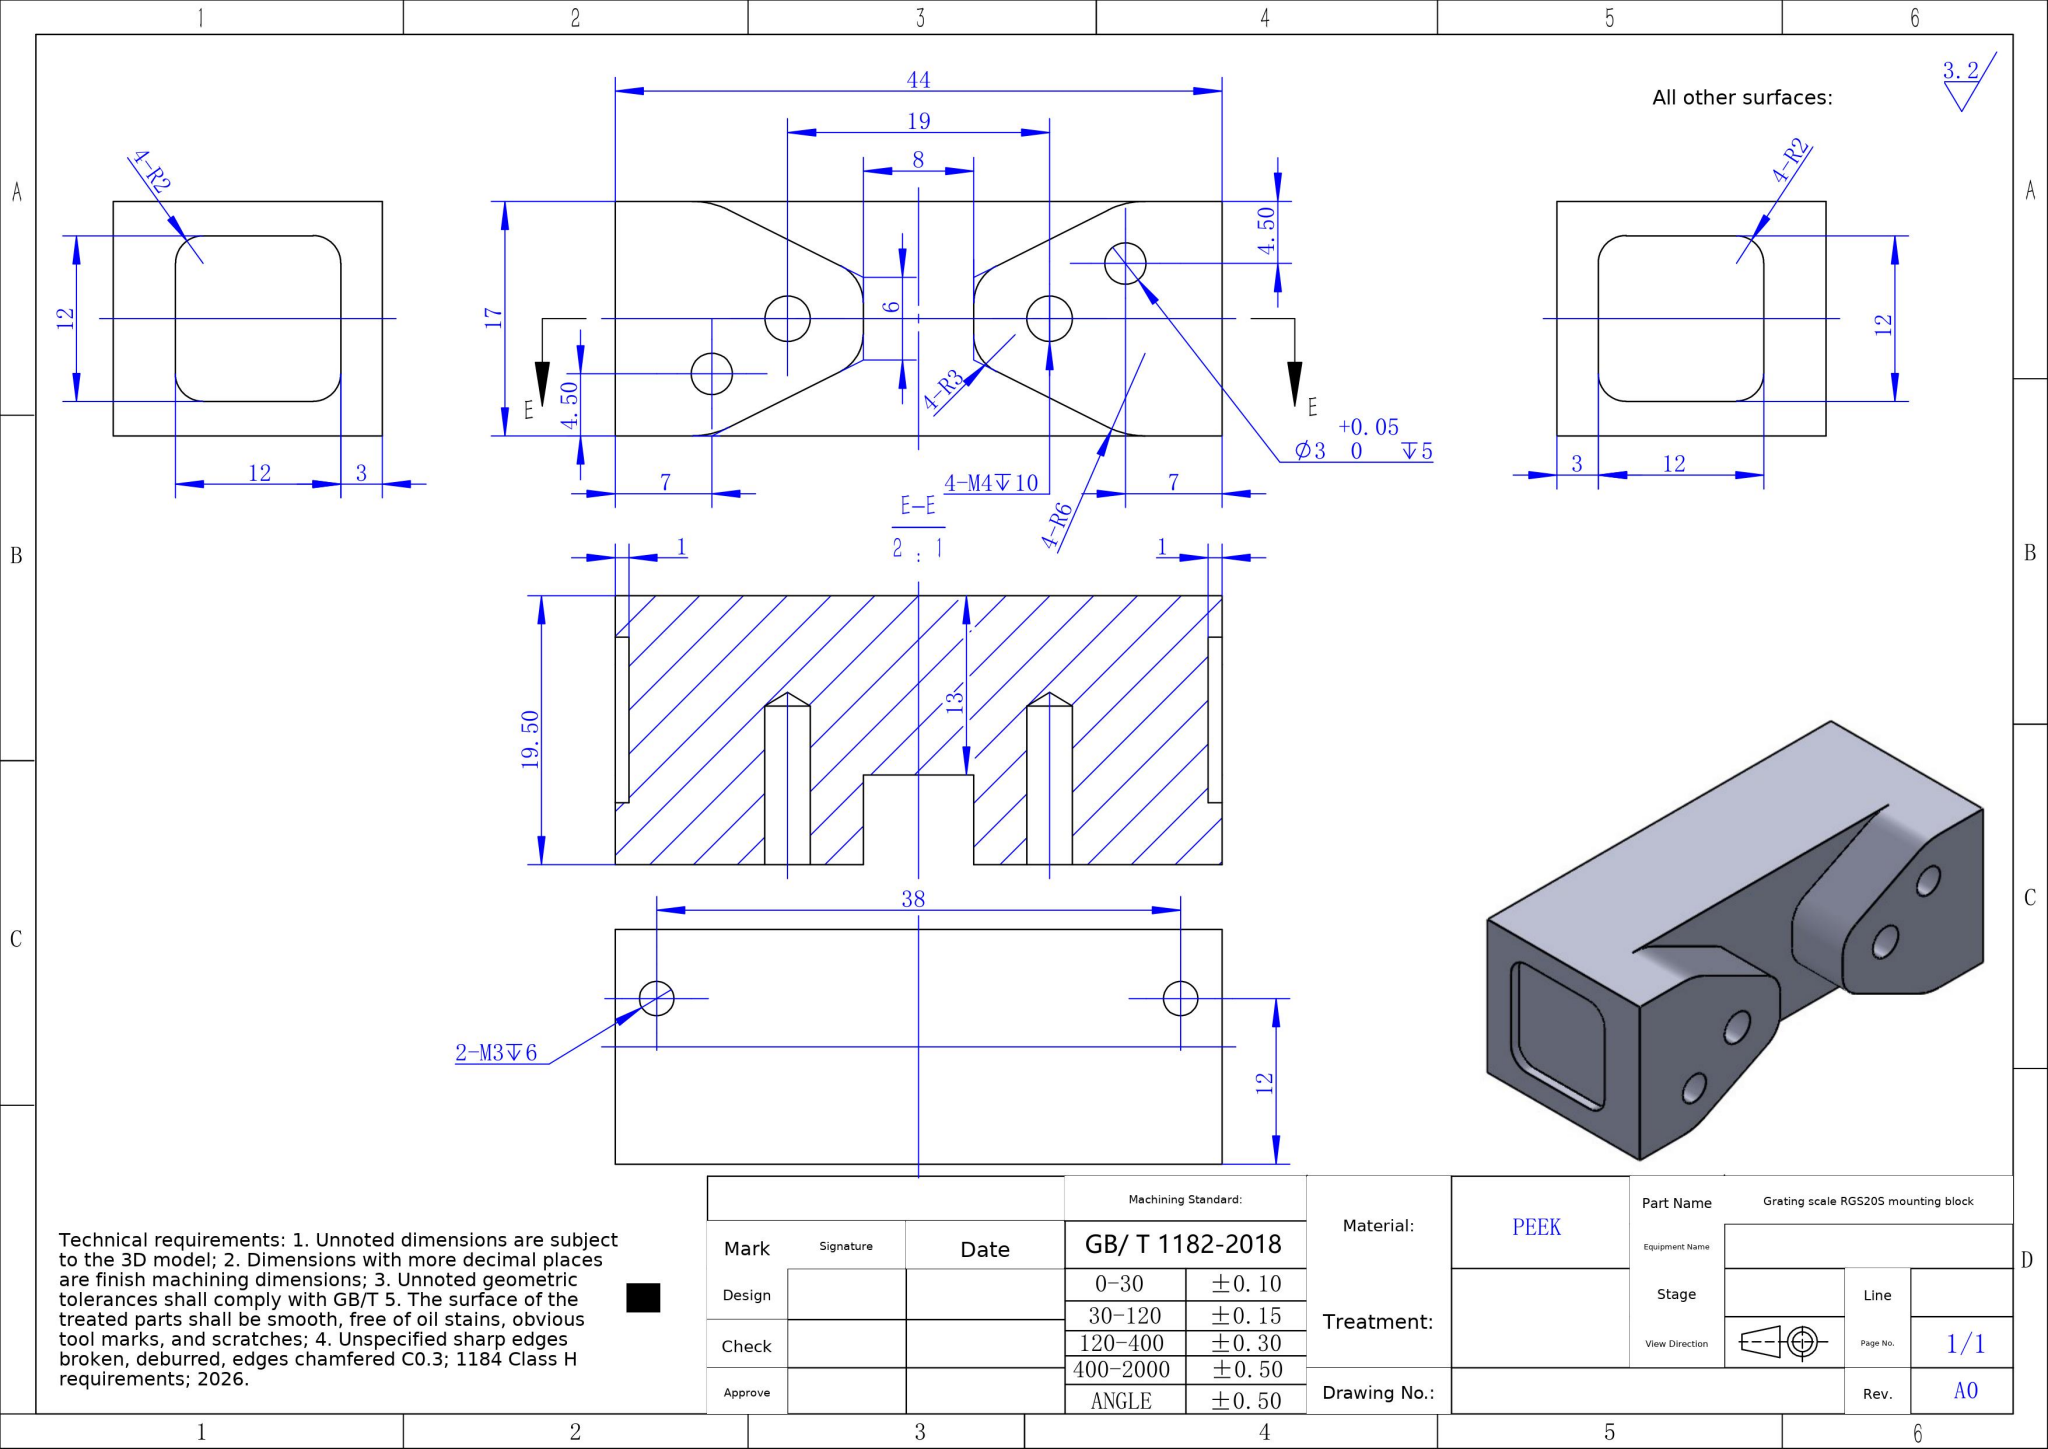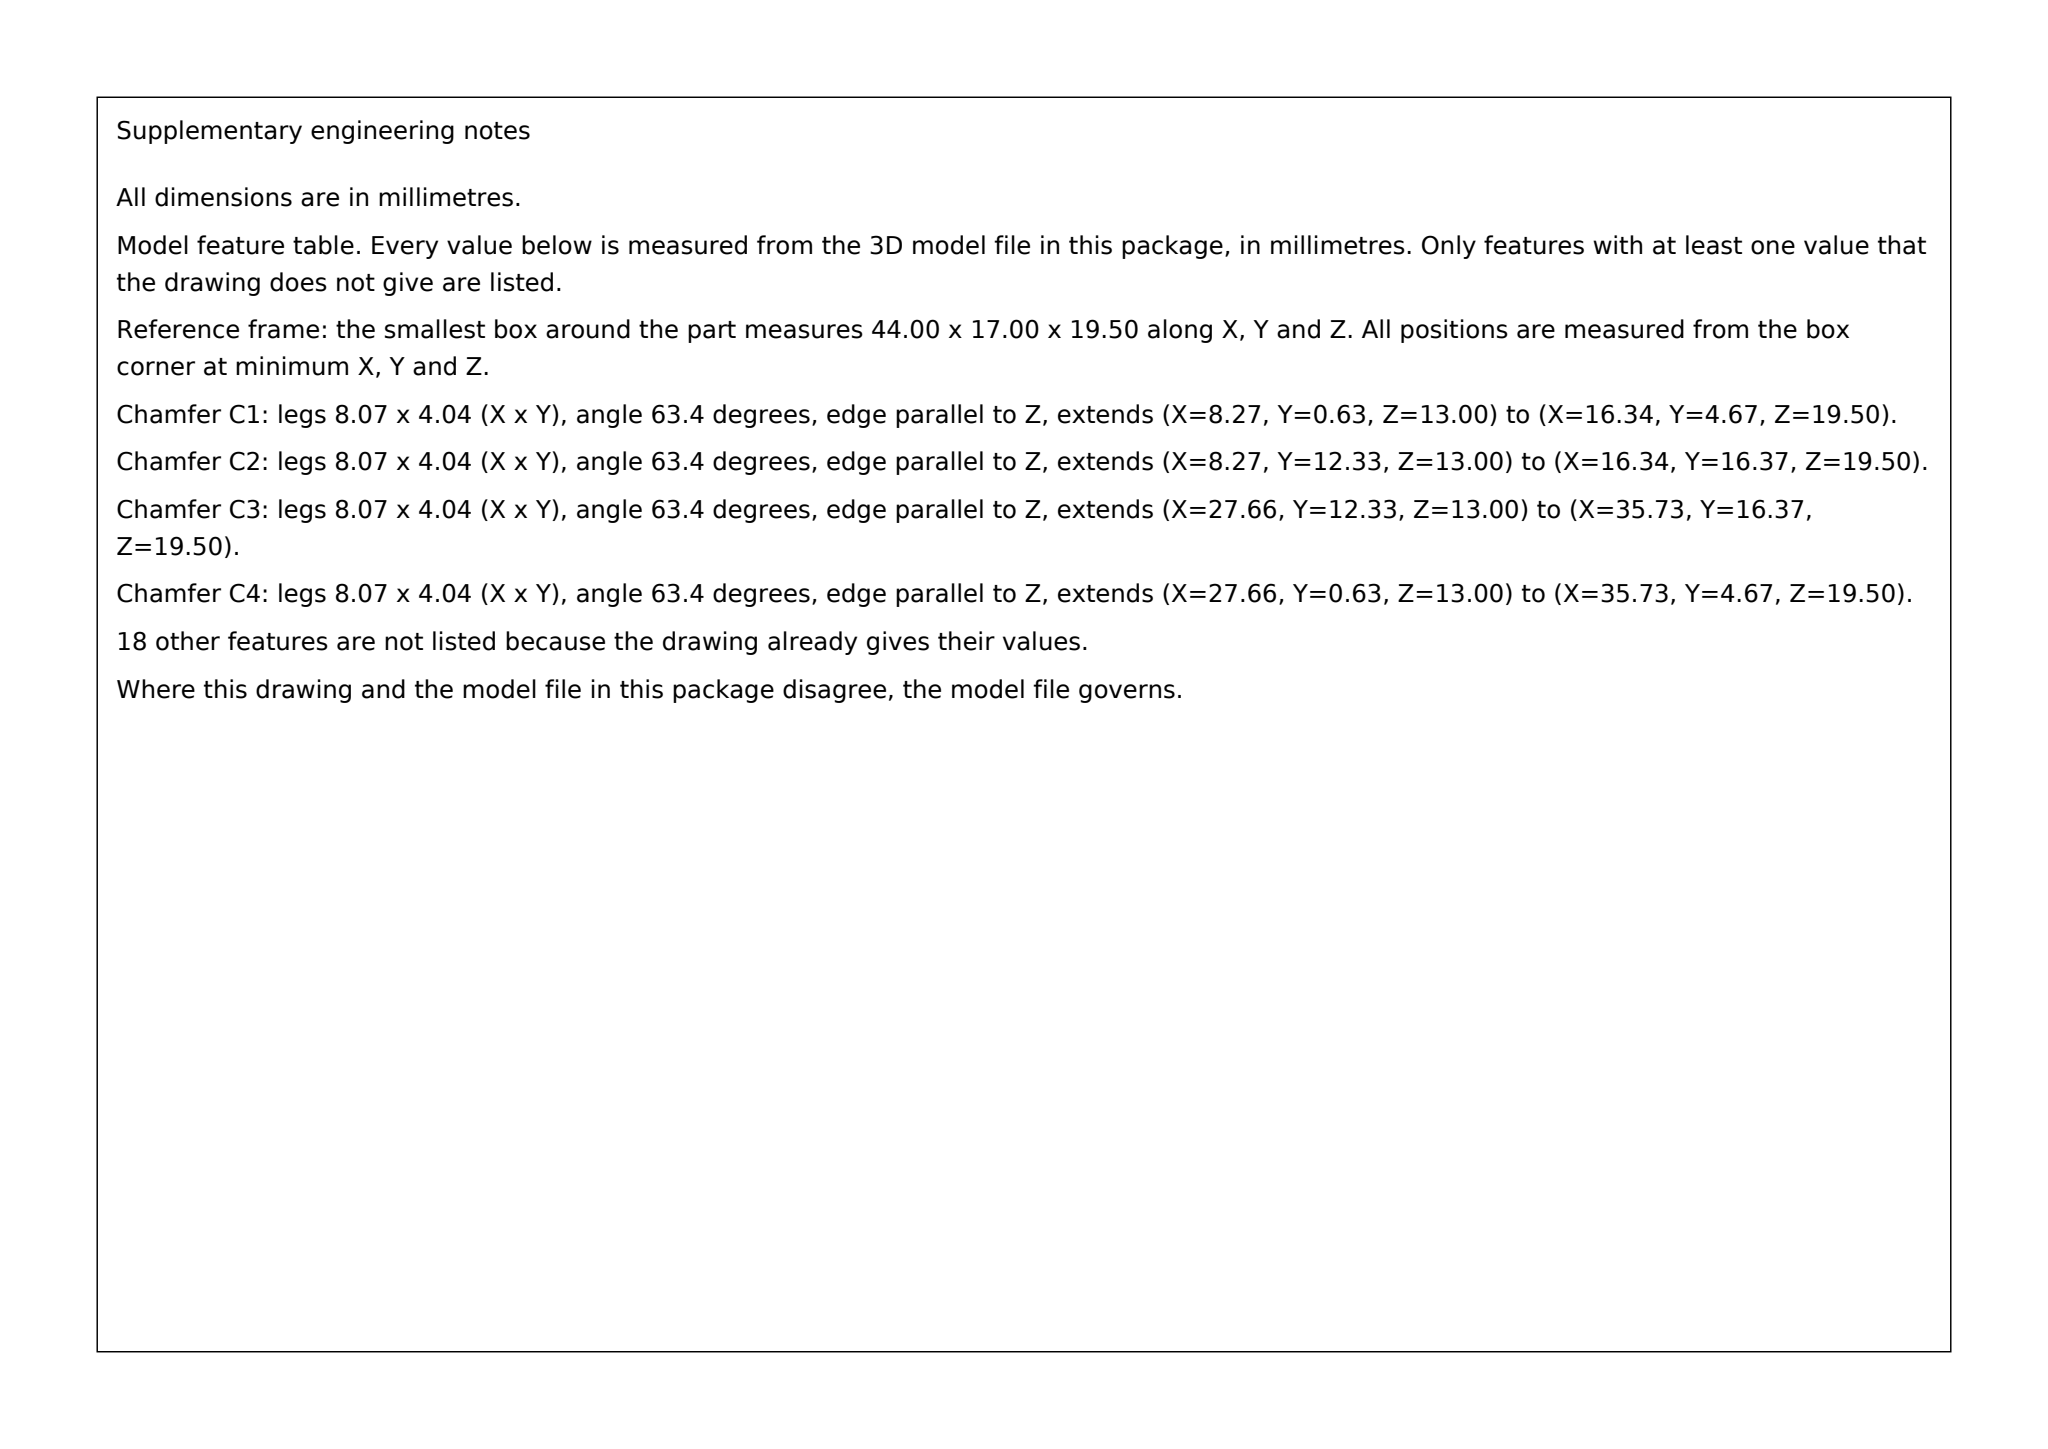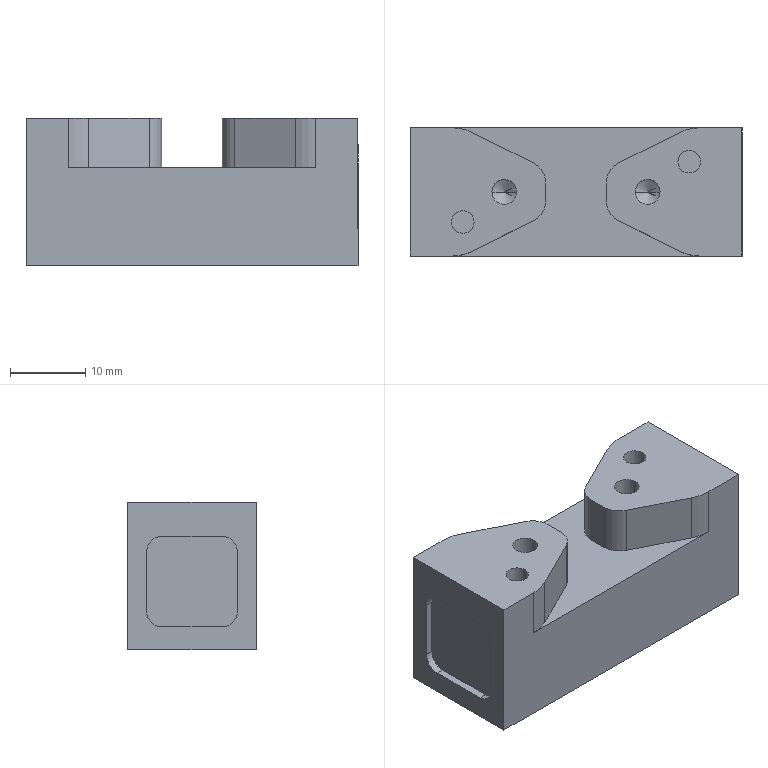Part | SolidWorks | mm | material PEEK | 1 solid | 62 faces | box 44 x 17 x 19.5 mm | volume 12256 mm3 | cylinder 28 | plane 26 | cone 8 | commonest cylinder face diameters 4 x8 3 x4 2.5 x4 3.3 x4 6 x4 12 x4